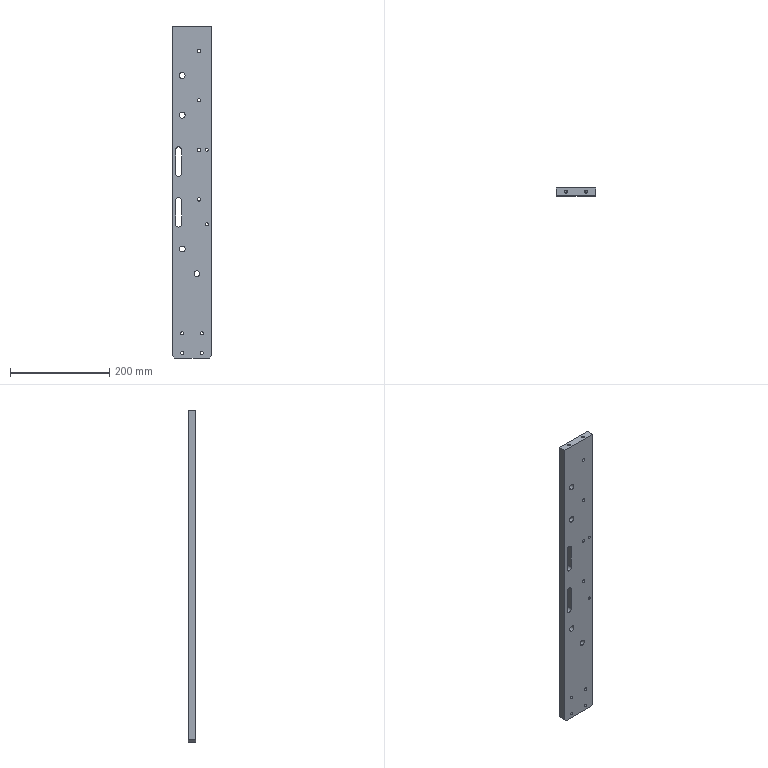Component | SolidWorks | 8TC-A15004-80-01A-1 | 1 solid | 66 faces | box 80 x 15 x 670 mm | volume 769310 mm3 | cylinder 46 | plane 16 | cone 4 | commonest cylinder face diameters 6 x16 12 x14 11 x8 6.6 x8 | material A3
build123d program:
from build123d import *

# Parameters (mm, degrees)
SKETCH1_W                                       = 80
SKETCH1_H                                       = 670
BOSS_EXTRUDE1_DEPTH                             = 7.5
SKETCH2_R                                       = 6
CUT_EXTRUDE1_DEPTH                              = 675.926
CHAMFER1_SIZE                                   = 5
M6_HEX_SOCKET_HEAD_CAP_SCREW_CBORE1_D           = 6.6
M6_HEX_SOCKET_HEAD_CAP_SCREW_CBORE1_CBORE_D     = 11
M6_HEX_SOCKET_HEAD_CAP_SCREW_CBORE1_CBORE_DEPTH = 6.4
M6_TAPPED_HOLE1_D                               = 6
M6_TAPPED_HOLE2_D                               = 6
M6_TAPPED_HOLE3_D                               = 6
M6_TAPPED_HOLE3_DEPTH                           = 15
M6_TAPPED_HOLE3_TIP                             = 1.803
CUT_EXTRUDE2_DEPTH                              = 675.926


with BuildPart() as part:
    # Sketch1 → Boss-Extrude1 (new, symmetric)
    with BuildSketch(Plane(origin=(0, 0, 0), x_dir=(1, 0, 0), z_dir=(0, 1, 0))):
        with Locations((40, 335)):
            Rectangle(SKETCH1_W, SKETCH1_H)
    extrude(amount=BOSS_EXTRUDE1_DEPTH, both=True)

    # Sketch2 → Cut-Extrude1 (cut, through all)
    with BuildSketch(Plane(origin=(0, 7.5, 0), x_dir=(1, 0, 0), z_dir=(0, 1, 0))):
        with Locations(Location((50, 500, 0), (0, 0, 270))):
            Circle(SKETCH2_R)
        with Locations(Location((20, 450, 0), (0, 0, 270))):
            Circle(SKETCH2_R)
        with Locations(Location((20, 180, 0), (0, 0, 90))):
            Circle(SKETCH2_R)
        with Locations(Location((20, 100, 0), (0, 0, 90))):
            Circle(SKETCH2_R)
    extrude(amount=-CUT_EXTRUDE1_DEPTH, mode=Mode.SUBTRACT)

    # Chamfer1
    chamfer1_edges = [part.edges().sort_by_distance(p)[0] for p in [
        (0, 0, -670),
        (80, 0, -670),
    ]]
    chamfer(chamfer1_edges, length=CHAMFER1_SIZE)

    # M6 Hex Socket Head Cap Screw CBORE1 (through all)
    with Locations(Plane(origin=(0, 7.5, 0), x_dir=(1, 0, 0), z_dir=(0, 1, 0))):
        with Locations((54, 50), (54, 150), (54, 250), (54, 350)):
            CounterBoreHole(M6_HEX_SOCKET_HEAD_CAP_SCREW_CBORE1_D / 2, M6_HEX_SOCKET_HEAD_CAP_SCREW_CBORE1_CBORE_D / 2, M6_HEX_SOCKET_HEAD_CAP_SCREW_CBORE1_CBORE_DEPTH)

    # M6 Tapped Hole1 (through all)
    with Locations(Plane(origin=(0, 7.5, 0), x_dir=(1, 0, 0), z_dir=(0, 1, 0))):
        with Locations((70, 400), (70, 250)):
            Hole(M6_TAPPED_HOLE1_D / 2)

    # M6 Tapped Hole2 (through all)
    with Locations(Plane(origin=(0, 7.5, 0), x_dir=(1, 0, 0), z_dir=(0, 1, 0))):
        with Locations((20, 620), (60, 620), (20, 660), (60, 660)):
            Hole(M6_TAPPED_HOLE2_D / 2)

    # M6 Tapped Hole3
    with Locations(Plane.XY):
        with Locations((20, 0), (60, 0)):
            Hole(M6_TAPPED_HOLE3_D / 2, depth=M6_TAPPED_HOLE3_DEPTH)
            with Locations((0, 0, -(M6_TAPPED_HOLE3_DEPTH + M6_TAPPED_HOLE3_TIP / 2))):  # 118° drill point
                Cone(0, M6_TAPPED_HOLE3_D / 2, M6_TAPPED_HOLE3_TIP, mode=Mode.SUBTRACT)

    # Sketch11 → Cut-Extrude2 (cut, through all)
    with BuildSketch(Plane(origin=(0, 7.5, 0), x_dir=(1, 0, 0), z_dir=(0, 1, 0))):
        with BuildLine():
            Line((7, 352.5), (7, 400))
            ThreePointArc((7, 400), (13, 406), (19, 400))
            Line((19, 400), (19, 352.5))
            ThreePointArc((19, 352.5), (13, 346.5), (7, 352.5))
        make_face()
        with BuildLine():
            Line((19, 297.5), (19, 250))
            ThreePointArc((19, 250), (13, 244), (7, 250))
            Line((7, 250), (7, 297.5))
            ThreePointArc((7, 297.5), (13, 303.5), (19, 297.5))
        make_face()
    extrude(amount=-CUT_EXTRUDE2_DEPTH, mode=Mode.SUBTRACT)


solid = part.part